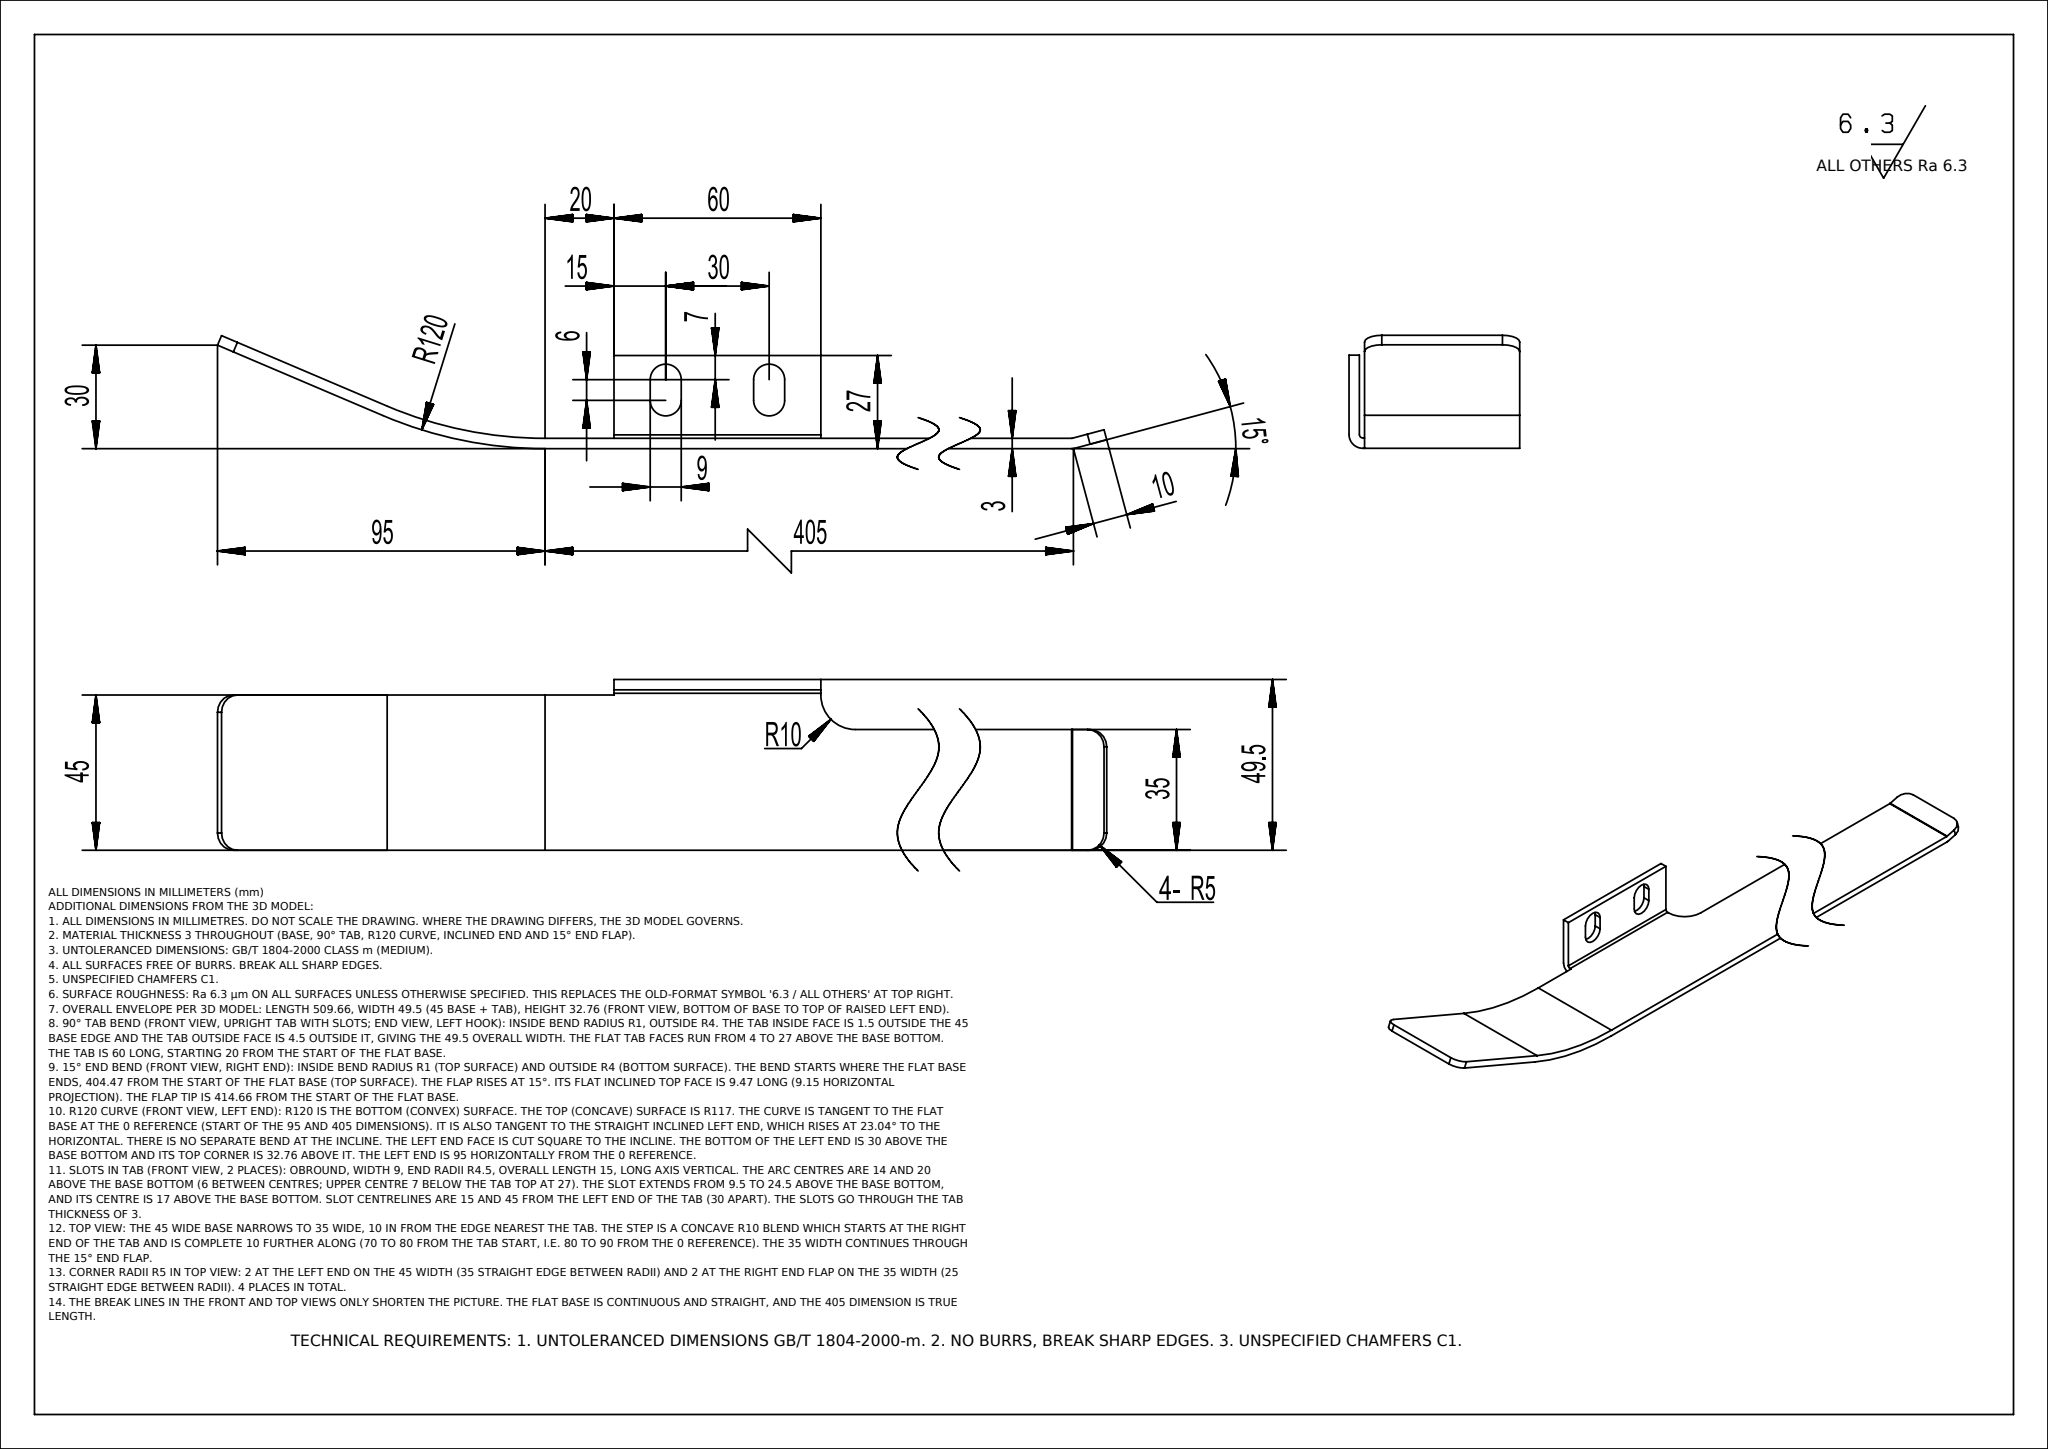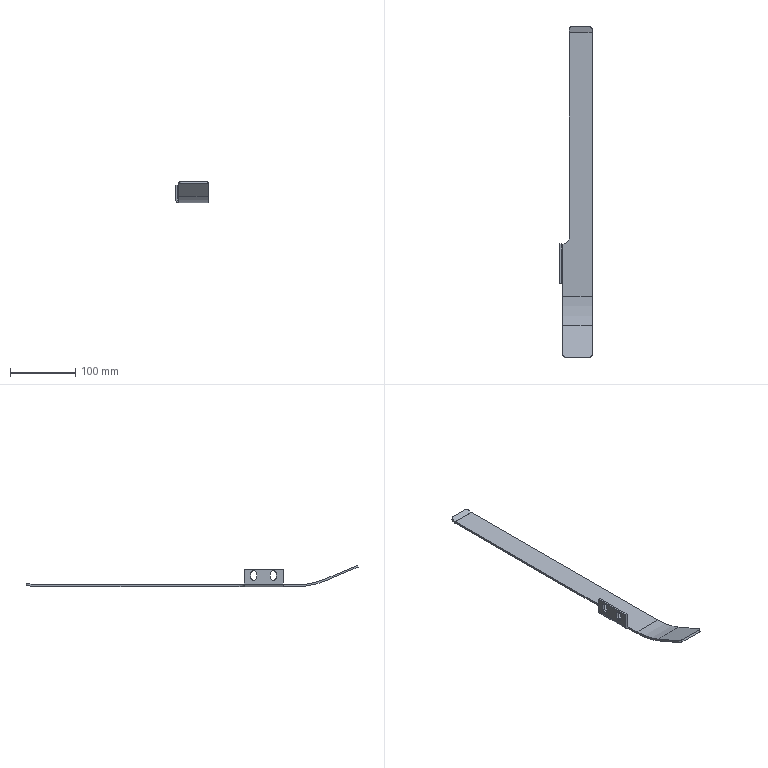Part | NX | mm | 1 solid | 35 faces | box 49.5 x 509.66 x 32.76 mm | volume 63644 mm3 | plane 20 | cylinder 15 | commonest cylinder face diameters 9 x4 10 x4 2 x2 8 x2 234 x1 240 x1 20 x1